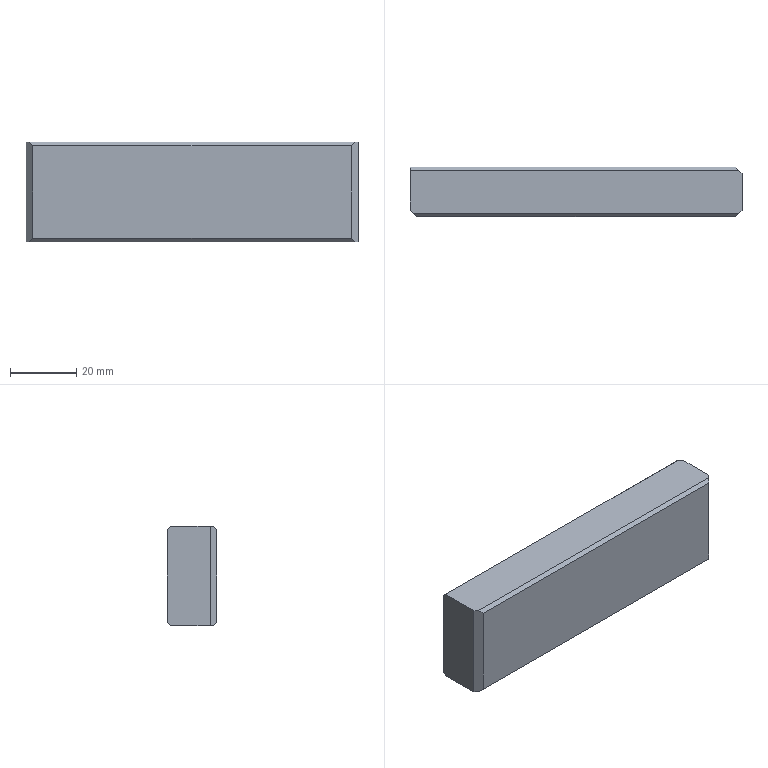Component | SolidWorks | 07.1.1-1 | 1 solid | 13 faces | box 100 x 15 x 30 mm | volume 44625 mm3 | plane 13
build123d program:
from build123d import *

# Parameters (mm, degrees)
SKETCH1_W           = 100
SKETCH1_H           = 30
BOSS_EXTRUDE1_DEPTH = 7.5
CHAMFER2_SIZE       = 2
CHAMFER3_SIZE       = 1


with BuildPart() as part:
    # Sketch1 → Boss-Extrude1 (new, symmetric)
    with BuildSketch(Plane.XY):
        Rectangle(SKETCH1_W, SKETCH1_H)
    extrude(amount=BOSS_EXTRUDE1_DEPTH, both=True)

    # Chamfer2
    chamfer2_edges = [part.edges().sort_by_distance(p)[0] for p in [
        (-50, 0, 7.5),
        (-50, 0, -7.5),
        (50, 0, -7.5),
    ]]
    chamfer(chamfer2_edges, length=CHAMFER2_SIZE)

    # Chamfer3
    chamfer3_edges = [part.edges().sort_by_distance(p)[0] for p in [
        (0, 15, -7.5),
        (0, -15, -7.5),
        (1, -15, 7.5),
        (1, 15, 7.5),
    ]]
    chamfer(chamfer3_edges, length=CHAMFER3_SIZE)


solid = part.part

# Placed as in the assembly
solid = solid.moved(Location((218.631, 1155.864, 173.477), (-90, 0, 180)))